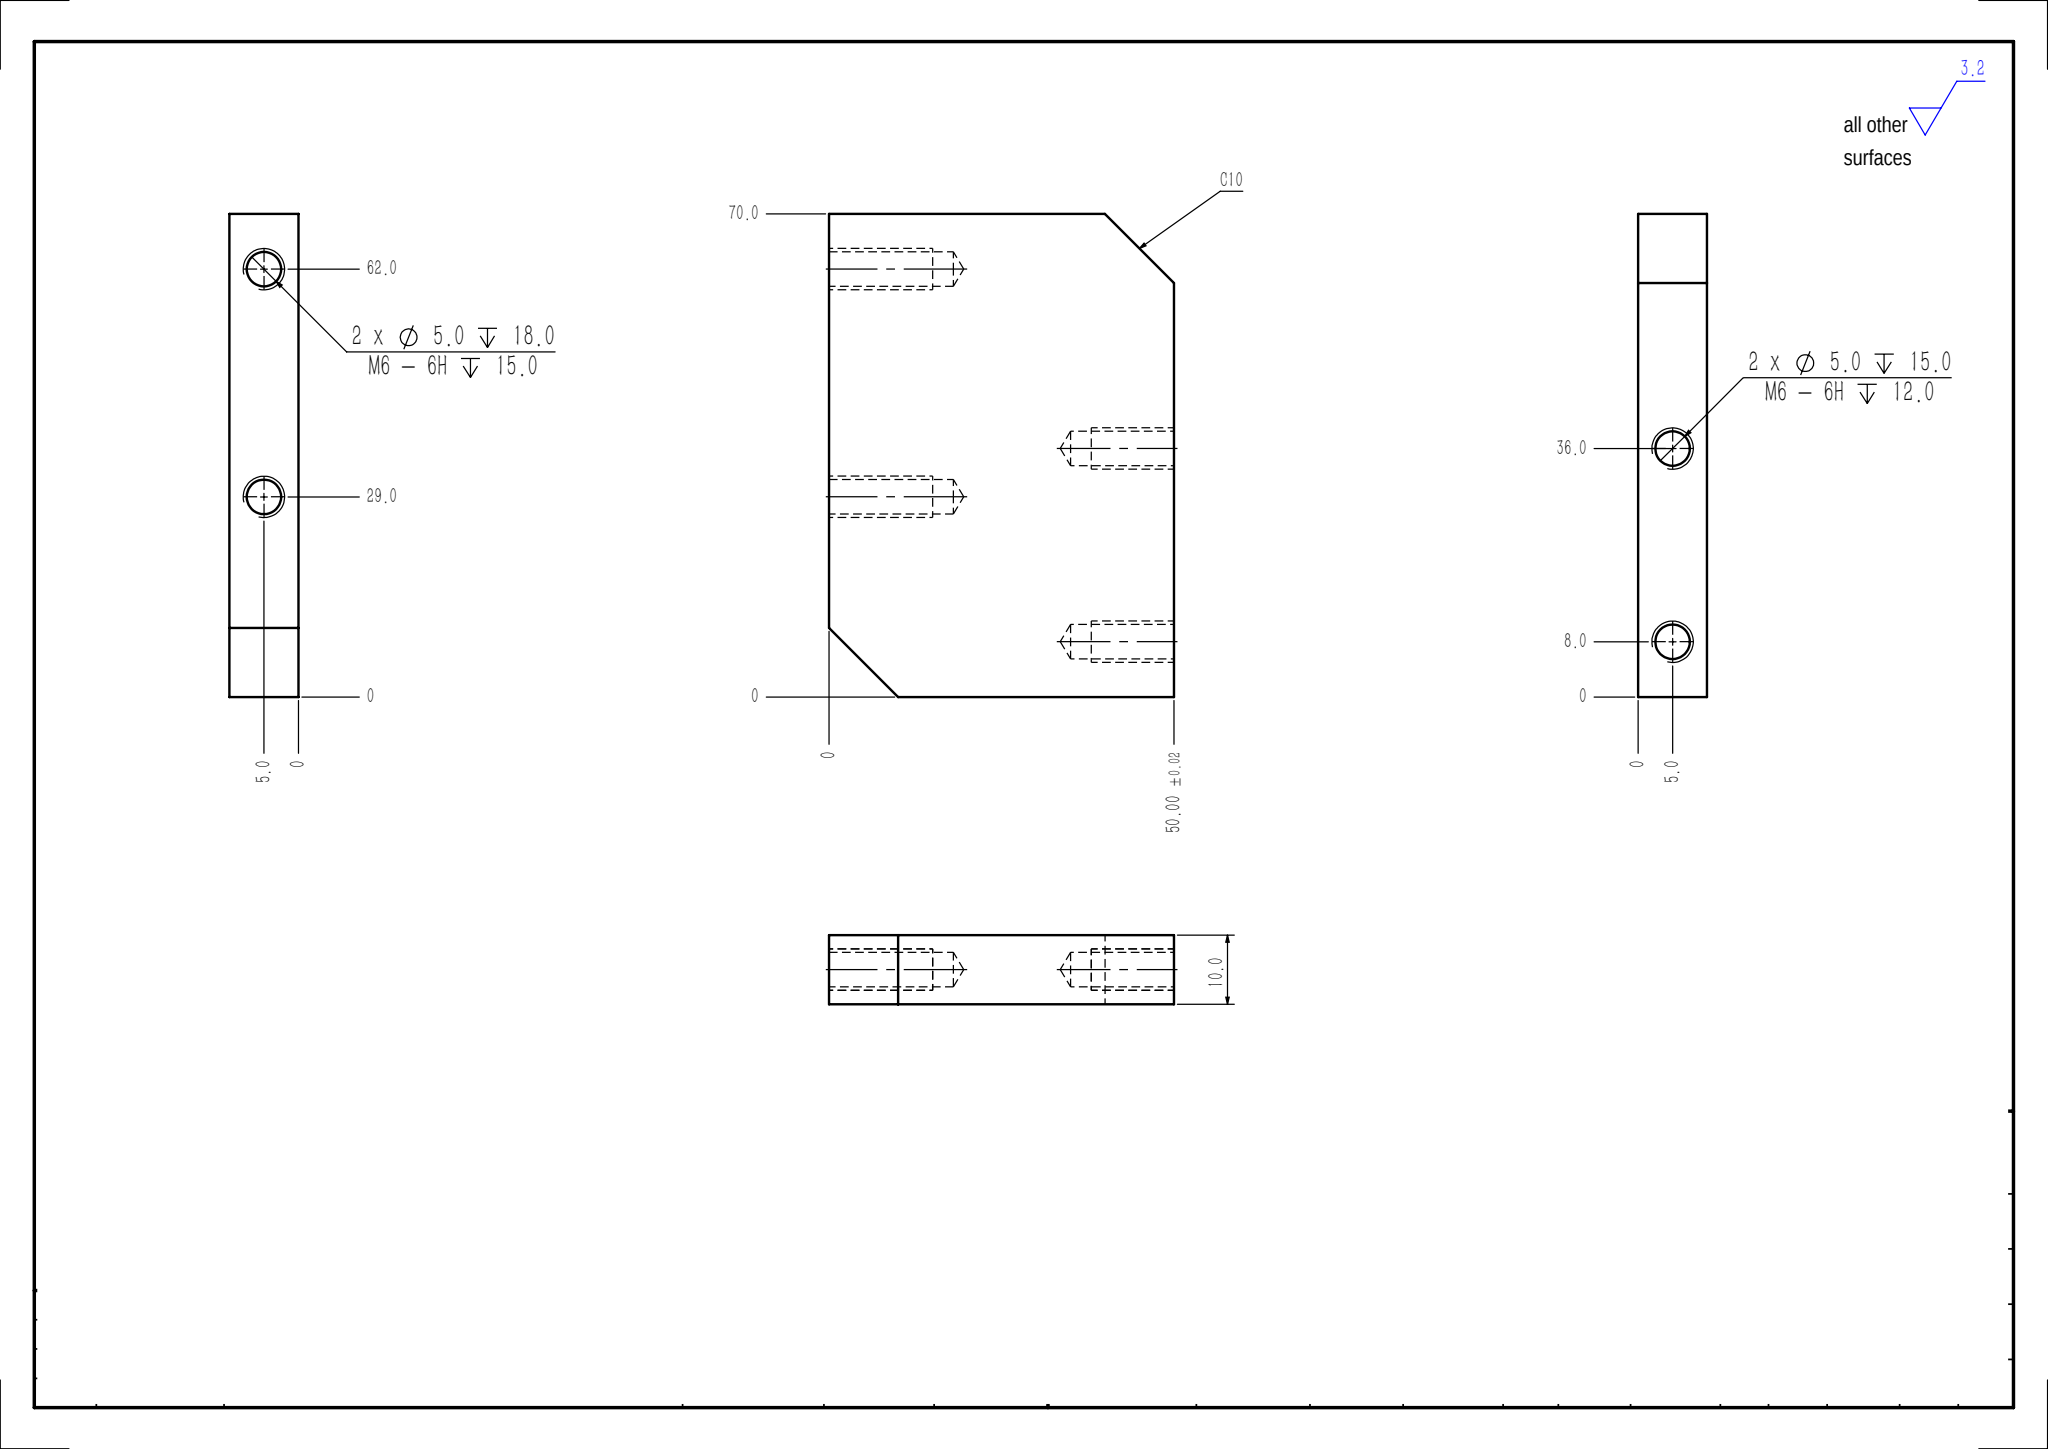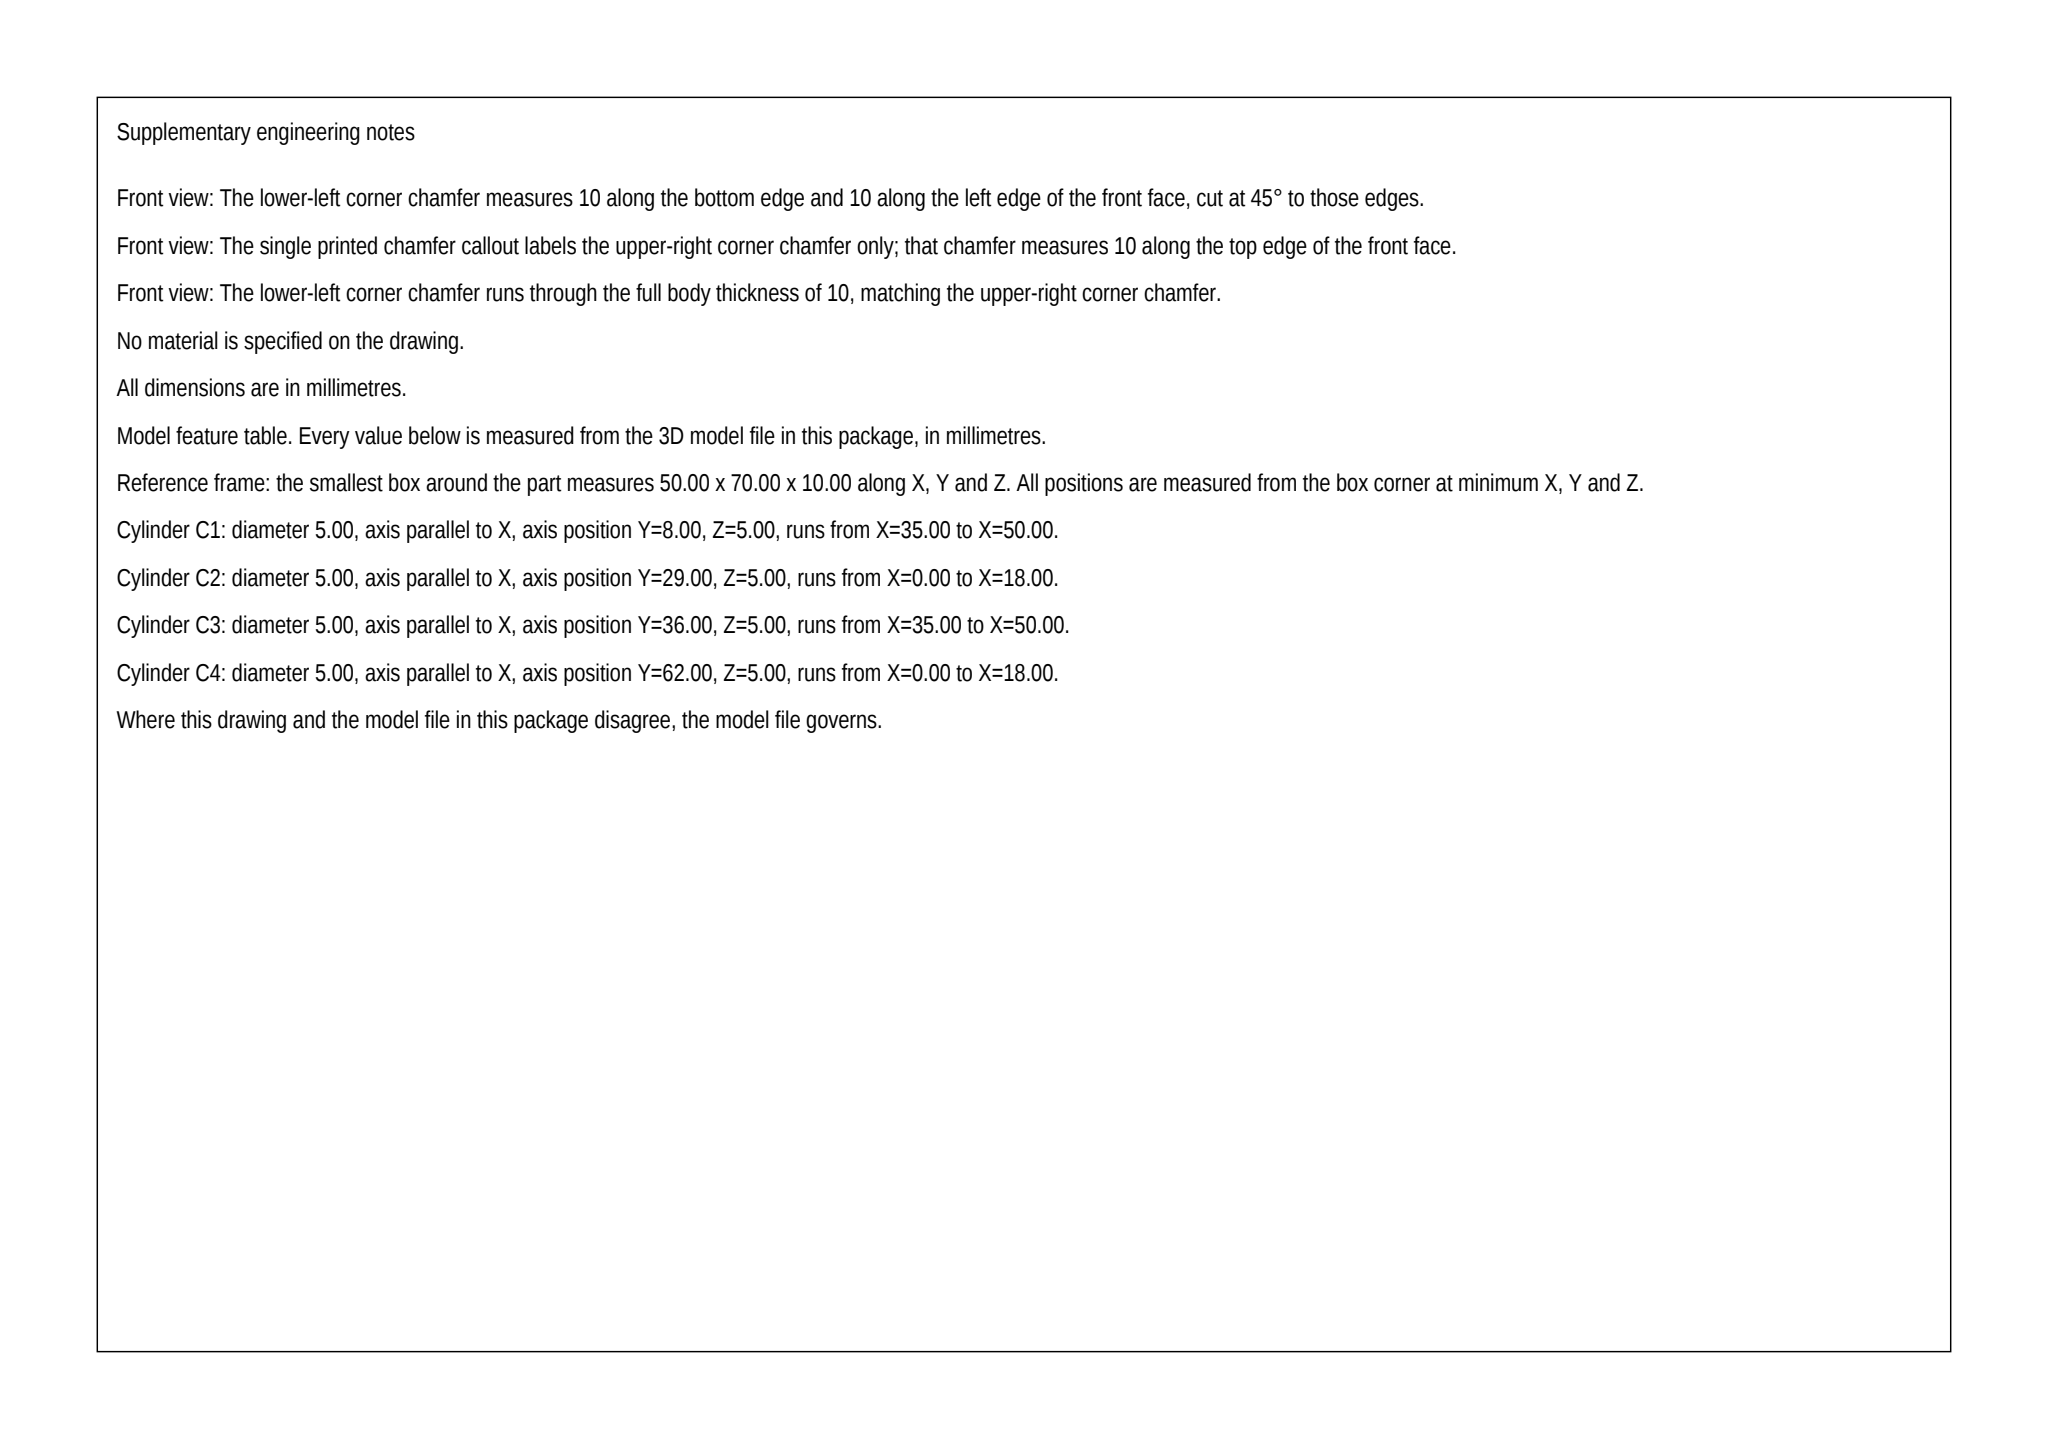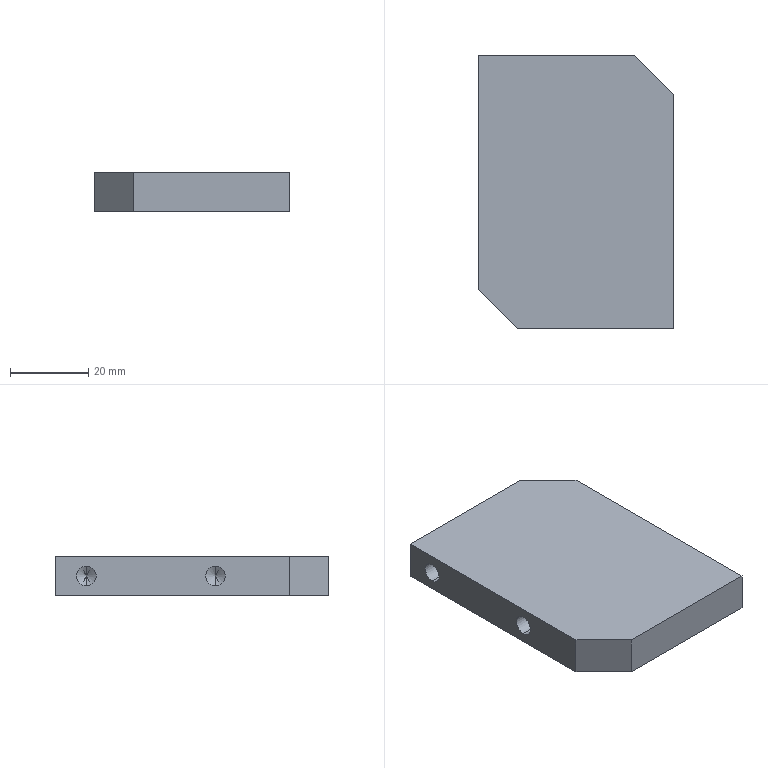Part | SolidWorks | mm | 1 solid | 24 faces | box 50 x 70 x 10 mm | volume 32665 mm3 | cylinder 8 | cone 8 | plane 8 | commonest cylinder face diameters 5 x8
Drawing notes:
C10 LOWER LEFT CORNER, FRONT VIEW (2X C10, 45 DEG) | from the solid: 50x70x10 bbox; lower-left corner cut 45 deg, 10 x 10 across corner, matching upper-right C10
2X C10 CHAMFER AT DIAG OPP CORNERS OF FRONT VIEW (TOP RH, BTM LH) | from the solid: inclined_planes: 45 deg faces, size 10x10x10, bbox_from [0,0,0] and [40,60,0] on 50x70x10 bbox
CHAMFERS FULL 10.0 THRU THICKNESS; NO OTHER CHAMFERS | from the solid: both inclined planes span z 0-10 (thickness 10.0); only 2 inclined planes in model
build123d program:
from build123d import *

# Parameters (mm, degrees)
SKETCH1_W             = 50
SKETCH1_H             = 70
BOSS_EXTRUDE1_DEPTH   = 10
M6_TAPPED_HOLE1_D     = 5
M6_TAPPED_HOLE1_DEPTH = 18
M6_TAPPED_HOLE1_TIP   = 1.502
M6_TAPPED_HOLE2_D     = 5
M6_TAPPED_HOLE2_DEPTH = 15
M6_TAPPED_HOLE2_TIP   = 1.502
CHAMFER1_SIZE         = 10


with BuildPart() as part:
    # Sketch1 → Boss-Extrude1 (new body)
    with BuildSketch(Plane.XY):
        Rectangle(SKETCH1_W, SKETCH1_H)
    extrude(amount=BOSS_EXTRUDE1_DEPTH)

    # M6 Tapped Hole1
    with Locations(Plane.ZY.offset(25)):
        with Locations((5, 27), (5, -6)):
            Hole(M6_TAPPED_HOLE1_D / 2, depth=M6_TAPPED_HOLE1_DEPTH)
            with Locations((0, 0, -(M6_TAPPED_HOLE1_DEPTH + M6_TAPPED_HOLE1_TIP / 2))):  # 118° drill point
                Cone(0, M6_TAPPED_HOLE1_D / 2, M6_TAPPED_HOLE1_TIP, mode=Mode.SUBTRACT)

    # M6 Tapped Hole2
    with Locations(Plane(origin=(25, 0, 0), x_dir=(0, 0, -1), z_dir=(1, 0, 0))):
        with Locations((-5, -27), (-5, 1)):
            Hole(M6_TAPPED_HOLE2_D / 2, depth=M6_TAPPED_HOLE2_DEPTH)
            with Locations((0, 0, -(M6_TAPPED_HOLE2_DEPTH + M6_TAPPED_HOLE2_TIP / 2))):  # 118° drill point
                Cone(0, M6_TAPPED_HOLE2_D / 2, M6_TAPPED_HOLE2_TIP, mode=Mode.SUBTRACT)

    # Chamfer1
    chamfer1_edges = [part.edges().sort_by_distance(p)[0] for p in [
        (-25, -35, 5),
        (25, 35, 5),
    ]]
    chamfer(chamfer1_edges, length=CHAMFER1_SIZE)


solid = part.part
STEP:
#1=CARTESIAN_POINT('',(10.,-27.,7.5));
#2=VERTEX_POINT('',#1);
#3=CARTESIAN_POINT('',(10.,-27.,2.5));
#4=VERTEX_POINT('',#3);
#5=CARTESIAN_POINT('',(10.,-27.,5.));
#6=DIRECTION('',(1.,0.,0.));
#7=DIRECTION('',(0.,0.,-1.));
#8=AXIS2_PLACEMENT_3D('',#5,#6,#7);
#9=CIRCLE('',#8,2.5);
#10=EDGE_CURVE('',#2,#4,#9,.T.);
#11=ORIENTED_EDGE('',*,*,#10,.F.);
#12=CARTESIAN_POINT('',(25.,-27.,7.5));
#13=VERTEX_POINT('',#12);
#14=CARTESIAN_POINT('',(25.,-27.,7.5));
#15=DIRECTION('',(1.,0.,0.));
#16=VECTOR('',#15,1000.);
#17=LINE('',#14,#16);
#18=EDGE_CURVE('',#2,#13,#17,.T.);
#19=ORIENTED_EDGE('',*,*,#18,.T.);
#20=CARTESIAN_POINT('',(25.,-27.,2.5));
#21=VERTEX_POINT('',#20);
#22=CARTESIAN_POINT('',(25.,-27.,5.));
#23=DIRECTION('',(1.,0.,0.));
#24=DIRECTION('',(0.,0.,-1.));
#25=AXIS2_PLACEMENT_3D('',#22,#23,#24);
#26=CIRCLE('',#25,2.5);
#27=EDGE_CURVE('',#13,#21,#26,.T.);
#28=ORIENTED_EDGE('',*,*,#27,.T.);
#29=CARTESIAN_POINT('',(25.,-27.,2.5));
#30=DIRECTION('',(1.,0.,0.));
#31=VECTOR('',#30,1000.);
#32=LINE('',#29,#31);
#33=EDGE_CURVE('',#4,#21,#32,.T.);
#34=ORIENTED_EDGE('',*,*,#33,.F.);
#35=EDGE_LOOP('',(#11,#19,#28,#34));
#36=FACE_OUTER_BOUND('',#35,.T.);
#37=CARTESIAN_POINT('',(25.,-27.,5.));
#38=DIRECTION('',(1.,0.,0.));
#39=DIRECTION('',(0.,0.,-1.));
#40=AXIS2_PLACEMENT_3D('',#37,#38,#39);
#41=CYLINDRICAL_SURFACE('',#40,2.5);
#42=ADVANCED_FACE('',(#36),#41,.F.);
#43=CARTESIAN_POINT('',(8.498,-27.,5.));
#44=VERTEX_POINT('',#43);
#45=CARTESIAN_POINT('',(10.,-27.,2.5));
#46=DIRECTION('',(0.515,0.,-0.8572));
#47=VECTOR('',#46,1000.);
#48=LINE('',#45,#47);
#49=EDGE_CURVE('',#44,#4,#48,.T.);
#50=ORIENTED_EDGE('',*,*,#49,.F.);
#51=CARTESIAN_POINT('',(10.,-27.,7.5));
#52=DIRECTION('',(0.515,0.,0.8572));
#53=VECTOR('',#52,1000.);
#54=LINE('',#51,#53);
#55=EDGE_CURVE('',#44,#2,#54,.T.);
#56=ORIENTED_EDGE('',*,*,#55,.T.);
#57=ORIENTED_EDGE('',*,*,#10,.T.);
#58=EDGE_LOOP('',(#50,#56,#57));
#59=FACE_OUTER_BOUND('',#58,.T.);
#60=CARTESIAN_POINT('',(10.,-27.,5.));
#61=DIRECTION('',(1.,0.,0.));
#62=DIRECTION('',(0.,0.,-1.));
#63=AXIS2_PLACEMENT_3D('',#60,#61,#62);
#64=CONICAL_SURFACE('',#63,2.5,1.03);
#65=ADVANCED_FACE('',(#59),#64,.F.);
#66=CARTESIAN_POINT('',(10.,1.,7.5));
#67=VERTEX_POINT('',#66);
#68=CARTESIAN_POINT('',(10.,1.,2.5));
#69=VERTEX_POINT('',#68);
#70=CARTESIAN_POINT('',(10.,1.,5.));
#71=DIRECTION('',(1.,0.,0.));
#72=DIRECTION('',(0.,0.,-1.));
#73=AXIS2_PLACEMENT_3D('',#70,#71,#72);
#74=CIRCLE('',#73,2.5);
#75=EDGE_CURVE('',#67,#69,#74,.T.);
#76=ORIENTED_EDGE('',*,*,#75,.F.);
#77=CARTESIAN_POINT('',(25.,1.,7.5));
#78=VERTEX_POINT('',#77);
#79=CARTESIAN_POINT('',(25.,1.,7.5));
#80=DIRECTION('',(1.,0.,0.));
#81=VECTOR('',#80,1000.);
#82=LINE('',#79,#81);
#83=EDGE_CURVE('',#67,#78,#82,.T.);
#84=ORIENTED_EDGE('',*,*,#83,.T.);
#85=CARTESIAN_POINT('',(25.,1.,2.5));
#86=VERTEX_POINT('',#85);
#87=CARTESIAN_POINT('',(25.,1.,5.));
#88=DIRECTION('',(1.,0.,0.));
#89=DIRECTION('',(0.,0.,-1.));
#90=AXIS2_PLACEMENT_3D('',#87,#88,#89);
#91=CIRCLE('',#90,2.5);
#92=EDGE_CURVE('',#78,#86,#91,.T.);
#93=ORIENTED_EDGE('',*,*,#92,.T.);
#94=CARTESIAN_POINT('',(25.,1.,2.5));
#95=DIRECTION('',(1.,0.,0.));
#96=VECTOR('',#95,1000.);
#97=LINE('',#94,#96);
#98=EDGE_CURVE('',#69,#86,#97,.T.);
#99=ORIENTED_EDGE('',*,*,#98,.F.);
#100=EDGE_LOOP('',(#76,#84,#93,#99));
#101=FACE_OUTER_BOUND('',#100,.T.);
#102=CARTESIAN_POINT('',(25.,1.,5.));
#103=DIRECTION('',(1.,0.,0.));
#104=DIRECTION('',(0.,0.,-1.));
#105=AXIS2_PLACEMENT_3D('',#102,#103,#104);
#106=CYLINDRICAL_SURFACE('',#105,2.5);
#107=ADVANCED_FACE('',(#101),#106,.F.);
#108=CARTESIAN_POINT('',(8.498,1.,5.));
#109=VERTEX_POINT('',#108);
#110=CARTESIAN_POINT('',(10.,1.,2.5));
#111=DIRECTION('',(0.515,0.,-0.8572));
#112=VECTOR('',#111,1000.);
#113=LINE('',#110,#112);
#114=EDGE_CURVE('',#109,#69,#113,.T.);
#115=ORIENTED_EDGE('',*,*,#114,.F.);
#116=CARTESIAN_POINT('',(10.,1.,7.5));
#117=DIRECTION('',(0.515,0.,0.8572));
#118=VECTOR('',#117,1000.);
#119=LINE('',#116,#118);
#120=EDGE_CURVE('',#109,#67,#119,.T.);
#121=ORIENTED_EDGE('',*,*,#120,.T.);
#122=ORIENTED_EDGE('',*,*,#75,.T.);
#123=EDGE_LOOP('',(#115,#121,#122));
#124=FACE_OUTER_BOUND('',#123,.T.);
#125=CARTESIAN_POINT('',(10.,1.,5.));
#126=DIRECTION('',(1.,0.,0.));
#127=DIRECTION('',(0.,0.,-1.));
#128=AXIS2_PLACEMENT_3D('',#125,#126,#127);
#129=CONICAL_SURFACE('',#128,2.5,1.03);
#130=ADVANCED_FACE('',(#124),#129,.F.);
#131=CARTESIAN_POINT('',(-7.,27.,2.5));
#132=VERTEX_POINT('',#131);
#133=CARTESIAN_POINT('',(-7.,27.,7.5));
#134=VERTEX_POINT('',#133);
#135=CARTESIAN_POINT('',(-7.,27.,5.));
#136=DIRECTION('',(-1.,0.,0.));
#137=DIRECTION('',(0.,0.,1.));
#138=AXIS2_PLACEMENT_3D('',#135,#136,#137);
#139=CIRCLE('',#138,2.5);
#140=EDGE_CURVE('',#132,#134,#139,.T.);
#141=ORIENTED_EDGE('',*,*,#140,.F.);
#142=CARTESIAN_POINT('',(-25.,27.,2.5));
#143=VERTEX_POINT('',#142);
#144=CARTESIAN_POINT('',(-25.,27.,2.5));
#145=DIRECTION('',(-1.,0.,0.));
#146=VECTOR('',#145,1000.);
#147=LINE('',#144,#146);
#148=EDGE_CURVE('',#132,#143,#147,.T.);
#149=ORIENTED_EDGE('',*,*,#148,.T.);
#150=CARTESIAN_POINT('',(-25.,27.,7.5));
#151=VERTEX_POINT('',#150);
#152=CARTESIAN_POINT('',(-25.,27.,5.));
#153=DIRECTION('',(-1.,0.,0.));
#154=DIRECTION('',(0.,0.,1.));
#155=AXIS2_PLACEMENT_3D('',#152,#153,#154);
#156=CIRCLE('',#155,2.5);
#157=EDGE_CURVE('',#143,#151,#156,.T.);
#158=ORIENTED_EDGE('',*,*,#157,.T.);
#159=CARTESIAN_POINT('',(-25.,27.,7.5));
#160=DIRECTION('',(-1.,0.,0.));
#161=VECTOR('',#160,1000.);
#162=LINE('',#159,#161);
#163=EDGE_CURVE('',#134,#151,#162,.T.);
#164=ORIENTED_EDGE('',*,*,#163,.F.);
#165=EDGE_LOOP('',(#141,#149,#158,#164));
#166=FACE_OUTER_BOUND('',#165,.T.);
#167=CARTESIAN_POINT('',(-25.,27.,5.));
#168=DIRECTION('',(-1.,0.,0.));
#169=DIRECTION('',(0.,0.,1.));
#170=AXIS2_PLACEMENT_3D('',#167,#168,#169);
#171=CYLINDRICAL_SURFACE('',#170,2.5);
#172=ADVANCED_FACE('',(#166),#171,.F.);
#173=CARTESIAN_POINT('',(-5.498,27.,5.));
#174=VERTEX_POINT('',#173);
#175=CARTESIAN_POINT('',(-7.,27.,7.5));
#176=DIRECTION('',(-0.515,0.,0.8572));
#177=VECTOR('',#176,1000.);
#178=LINE('',#175,#177);
#179=EDGE_CURVE('',#174,#134,#178,.T.);
#180=ORIENTED_EDGE('',*,*,#179,.F.);
#181=CARTESIAN_POINT('',(-7.,27.,2.5));
#182=DIRECTION('',(-0.515,0.,-0.8572));
#183=VECTOR('',#182,1000.);
#184=LINE('',#181,#183);
#185=EDGE_CURVE('',#174,#132,#184,.T.);
#186=ORIENTED_EDGE('',*,*,#185,.T.);
#187=ORIENTED_EDGE('',*,*,#140,.T.);
#188=EDGE_LOOP('',(#180,#186,#187));
#189=FACE_OUTER_BOUND('',#188,.T.);
#190=CARTESIAN_POINT('',(-7.,27.,5.));
#191=DIRECTION('',(-1.,0.,0.));
#192=DIRECTION('',(0.,0.,1.));
#193=AXIS2_PLACEMENT_3D('',#190,#191,#192);
#194=CONICAL_SURFACE('',#193,2.5,1.03);
#195=ADVANCED_FACE('',(#189),#194,.F.);
#196=CARTESIAN_POINT('',(-7.,-6.,2.5));
#197=VERTEX_POINT('',#196);
#198=CARTESIAN_POINT('',(-7.,-6.,7.5));
#199=VERTEX_POINT('',#198);
#200=CARTESIAN_POINT('',(-7.,-6.,5.));
#201=DIRECTION('',(-1.,0.,0.));
#202=DIRECTION('',(0.,0.,1.));
#203=AXIS2_PLACEMENT_3D('',#200,#201,#202);
#204=CIRCLE('',#203,2.5);
#205=EDGE_CURVE('',#197,#199,#204,.T.);
#206=ORIENTED_EDGE('',*,*,#205,.F.);
#207=CARTESIAN_POINT('',(-25.,-6.,2.5));
#208=VERTEX_POINT('',#207);
#209=CARTESIAN_POINT('',(-25.,-6.,2.5));
#210=DIRECTION('',(-1.,0.,0.));
#211=VECTOR('',#210,1000.);
#212=LINE('',#209,#211);
#213=EDGE_CURVE('',#197,#208,#212,.T.);
#214=ORIENTED_EDGE('',*,*,#213,.T.);
#215=CARTESIAN_POINT('',(-25.,-6.,7.5));
#216=VERTEX_POINT('',#215);
#217=CARTESIAN_POINT('',(-25.,-6.,5.));
#218=DIRECTION('',(-1.,0.,0.));
#219=DIRECTION('',(0.,0.,1.));
#220=AXIS2_PLACEMENT_3D('',#217,#218,#219);
#221=CIRCLE('',#220,2.5);
#222=EDGE_CURVE('',#208,#216,#221,.T.);
#223=ORIENTED_EDGE('',*,*,#222,.T.);
#224=CARTESIAN_POINT('',(-25.,-6.,7.5));
#225=DIRECTION('',(-1.,0.,0.));
#226=VECTOR('',#225,1000.);
#227=LINE('',#224,#226);
#228=EDGE_CURVE('',#199,#216,#227,.T.);
#229=ORIENTED_EDGE('',*,*,#228,.F.);
#230=EDGE_LOOP('',(#206,#214,#223,#229));
#231=FACE_OUTER_BOUND('',#230,.T.);
#232=CARTESIAN_POINT('',(-25.,-6.,5.));
#233=DIRECTION('',(-1.,0.,0.));
#234=DIRECTION('',(0.,0.,1.));
#235=AXIS2_PLACEMENT_3D('',#232,#233,#234);
#236=CYLINDRICAL_SURFACE('',#235,2.5);
#237=ADVANCED_FACE('',(#231),#236,.F.);
#238=CARTESIAN_POINT('',(-5.498,-6.,5.));
#239=VERTEX_POINT('',#238);
#240=CARTESIAN_POINT('',(-7.,-6.,7.5));
#241=DIRECTION('',(-0.515,0.,0.8572));
#242=VECTOR('',#241,1000.);
#243=LINE('',#240,#242);
#244=EDGE_CURVE('',#239,#199,#243,.T.);
#245=ORIENTED_EDGE('',*,*,#244,.F.);
#246=CARTESIAN_POINT('',(-7.,-6.,2.5));
#247=DIRECTION('',(-0.515,0.,-0.8572));
#248=VECTOR('',#247,1000.);
#249=LINE('',#246,#248);
#250=EDGE_CURVE('',#239,#197,#249,.T.);
#251=ORIENTED_EDGE('',*,*,#250,.T.);
#252=ORIENTED_EDGE('',*,*,#205,.T.);
#253=EDGE_LOOP('',(#245,#251,#252));
#254=FACE_OUTER_BOUND('',#253,.T.);
#255=CARTESIAN_POINT('',(-7.,-6.,5.));
#256=DIRECTION('',(-1.,0.,0.));
#257=DIRECTION('',(0.,0.,1.));
#258=AXIS2_PLACEMENT_3D('',#255,#256,#257);
#259=CONICAL_SURFACE('',#258,2.5,1.03);
#260=ADVANCED_FACE('',(#254),#259,.F.);
#261=CARTESIAN_POINT('',(25.,-27.,5.));
#262=DIRECTION('',(1.,0.,0.));
#263=DIRECTION('',(0.,0.,-1.));
#264=AXIS2_PLACEMENT_3D('',#261,#262,#263);
#265=CIRCLE('',#264,2.5);
#266=EDGE_CURVE('',#21,#13,#265,.T.);
#267=ORIENTED_EDGE('',*,*,#266,.F.);
#268=ORIENTED_EDGE('',*,*,#27,.F.);
#269=EDGE_LOOP('',(#267,#268));
#270=FACE_BOUND('',#269,.T.);
#271=CARTESIAN_POINT('',(25.,1.,5.));
#272=DIRECTION('',(1.,0.,0.));
#273=DIRECTION('',(0.,0.,-1.));
#274=AXIS2_PLACEMENT_3D('',#271,#272,#273);
#275=CIRCLE('',#274,2.5);
#276=EDGE_CURVE('',#86,#78,#275,.T.);
#277=ORIENTED_EDGE('',*,*,#276,.F.);
#278=ORIENTED_EDGE('',*,*,#92,.F.);
#279=EDGE_LOOP('',(#277,#278));
#280=FACE_BOUND('',#279,.T.);
#281=CARTESIAN_POINT('',(25.,-35.,0.));
#282=VERTEX_POINT('',#281);
#283=CARTESIAN_POINT('',(25.,25.,0.));
#284=VERTEX_POINT('',#283);
#285=CARTESIAN_POINT('',(25.,35.,0.));
#286=DIRECTION('',(-0.,1.,0.));
#287=VECTOR('',#286,1000.);
#288=LINE('',#285,#287);
#289=EDGE_CURVE('',#282,#284,#288,.T.);
#290=ORIENTED_EDGE('',*,*,#289,.T.);
#291=CARTESIAN_POINT('',(25.,25.,10.));
#292=VERTEX_POINT('',#291);
#293=CARTESIAN_POINT('',(25.,25.,10.));
#294=DIRECTION('',(0.,0.,1.));
#295=VECTOR('',#294,1000.);
#296=LINE('',#293,#295);
#297=EDGE_CURVE('',#284,#292,#296,.T.);
#298=ORIENTED_EDGE('',*,*,#297,.T.);
#299=CARTESIAN_POINT('',(25.,-35.,10.));
#300=VERTEX_POINT('',#299);
#301=CARTESIAN_POINT('',(25.,35.,10.));
#302=DIRECTION('',(-0.,1.,0.));
#303=VECTOR('',#302,1000.);
#304=LINE('',#301,#303);
#305=EDGE_CURVE('',#300,#292,#304,.T.);
#306=ORIENTED_EDGE('',*,*,#305,.F.);
#307=CARTESIAN_POINT('',(25.,-35.,10.));
#308=DIRECTION('',(0.,0.,-1.));
#309=VECTOR('',#308,1000.);
#310=LINE('',#307,#309);
#311=EDGE_CURVE('',#300,#282,#310,.T.);
#312=ORIENTED_EDGE('',*,*,#311,.T.);
#313=EDGE_LOOP('',(#290,#298,#306,#312));
#314=FACE_OUTER_BOUND('',#313,.T.);
#315=CARTESIAN_POINT('',(25.,35.,10.));
#316=DIRECTION('',(-1.,-0.,0.));
#317=DIRECTION('',(0.,-1.,0.));
#318=AXIS2_PLACEMENT_3D('',#315,#316,#317);
#319=PLANE('',#318);
#320=ADVANCED_FACE('',(#270,#280,#314),#319,.F.);
#321=CARTESIAN_POINT('',(15.,35.,10.));
#322=VERTEX_POINT('',#321);
#323=CARTESIAN_POINT('',(-25.,35.,10.));
#324=VERTEX_POINT('',#323);
#325=CARTESIAN_POINT('',(-25.,35.,10.));
#326=DIRECTION('',(-1.,0.,0.));
#327=VECTOR('',#326,1000.);
#328=LINE('',#325,#327);
#329=EDGE_CURVE('',#322,#324,#328,.T.);
#330=ORIENTED_EDGE('',*,*,#329,.F.);
#331=CARTESIAN_POINT('',(15.,35.,0.));
#332=VERTEX_POINT('',#331);
#333=CARTESIAN_POINT('',(15.,35.,10.));
#334=DIRECTION('',(0.,0.,-1.));
#335=VECTOR('',#334,1000.);
#336=LINE('',#333,#335);
#337=EDGE_CURVE('',#322,#332,#336,.T.);
#338=ORIENTED_EDGE('',*,*,#337,.T.);
#339=CARTESIAN_POINT('',(-25.,35.,0.));
#340=VERTEX_POINT('',#339);
#341=CARTESIAN_POINT('',(-25.,35.,0.));
#342=DIRECTION('',(-1.,0.,0.));
#343=VECTOR('',#342,1000.);
#344=LINE('',#341,#343);
#345=EDGE_CURVE('',#332,#340,#344,.T.);
#346=ORIENTED_EDGE('',*,*,#345,.T.);
#347=CARTESIAN_POINT('',(-25.,35.,10.));
#348=DIRECTION('',(0.,0.,-1.));
#349=VECTOR('',#348,1000.);
#350=LINE('',#347,#349);
#351=EDGE_CURVE('',#324,#340,#350,.T.);
#352=ORIENTED_EDGE('',*,*,#351,.F.);
#353=EDGE_LOOP('',(#330,#338,#346,#352));
#354=FACE_OUTER_BOUND('',#353,.T.);
#355=CARTESIAN_POINT('',(-25.,35.,10.));
#356=DIRECTION('',(0.,-1.,0.));
#357=DIRECTION('',(0.,0.,-1.));
#358=AXIS2_PLACEMENT_3D('',#355,#356,#357);
#359=PLANE('',#358);
#360=ADVANCED_FACE('',(#354),#359,.F.);
#361=CARTESIAN_POINT('',(-25.,27.,5.));
#362=DIRECTION('',(-1.,0.,0.));
#363=DIRECTION('',(0.,0.,1.));
#364=AXIS2_PLACEMENT_3D('',#361,#362,#363);
#365=CIRCLE('',#364,2.5);
#366=EDGE_CURVE('',#151,#143,#365,.T.);
#367=ORIENTED_EDGE('',*,*,#366,.F.);
#368=ORIENTED_EDGE('',*,*,#157,.F.);
#369=EDGE_LOOP('',(#367,#368));
#370=FACE_BOUND('',#369,.T.);
#371=CARTESIAN_POINT('',(-25.,-6.,5.));
#372=DIRECTION('',(-1.,0.,0.));
#373=DIRECTION('',(0.,0.,1.));
#374=AXIS2_PLACEMENT_3D('',#371,#372,#373);
#375=CIRCLE('',#374,2.5);
#376=EDGE_CURVE('',#216,#208,#375,.T.);
#377=ORIENTED_EDGE('',*,*,#376,.F.);
#378=ORIENTED_EDGE('',*,*,#222,.F.);
#379=EDGE_LOOP('',(#377,#378));
#380=FACE_BOUND('',#379,.T.);
#381=CARTESIAN_POINT('',(-25.,-25.,0.));
#382=VERTEX_POINT('',#381);
#383=CARTESIAN_POINT('',(-25.,35.,0.));
#384=DIRECTION('',(0.,-1.,0.));
#385=VECTOR('',#384,1000.);
#386=LINE('',#383,#385);
#387=EDGE_CURVE('',#340,#382,#386,.T.);
#388=ORIENTED_EDGE('',*,*,#387,.T.);
#389=CARTESIAN_POINT('',(-25.,-25.,10.));
#390=VERTEX_POINT('',#389);
#391=CARTESIAN_POINT('',(-25.,-25.,10.));
#392=DIRECTION('',(0.,0.,1.));
#393=VECTOR('',#392,1000.);
#394=LINE('',#391,#393);
#395=EDGE_CURVE('',#382,#390,#394,.T.);
#396=ORIENTED_EDGE('',*,*,#395,.T.);
#397=CARTESIAN_POINT('',(-25.,35.,10.));
#398=DIRECTION('',(0.,-1.,0.));
#399=VECTOR('',#398,1000.);
#400=LINE('',#397,#399);
#401=EDGE_CURVE('',#324,#390,#400,.T.);
#402=ORIENTED_EDGE('',*,*,#401,.F.);
#403=ORIENTED_EDGE('',*,*,#351,.T.);
#404=EDGE_LOOP('',(#388,#396,#402,#403));
#405=FACE_OUTER_BOUND('',#404,.T.);
#406=CARTESIAN_POINT('',(-25.,35.,10.));
#407=DIRECTION('',(1.,0.,0.));
#408=DIRECTION('',(-0.,1.,0.));
#409=AXIS2_PLACEMENT_3D('',#406,#407,#408);
#410=PLANE('',#409);
#411=ADVANCED_FACE('',(#370,#380,#405),#410,.F.);
#412=CARTESIAN_POINT('',(-15.,-35.,10.));
#413=VERTEX_POINT('',#412);
#414=CARTESIAN_POINT('',(-25.,-35.,10.));
#415=DIRECTION('',(1.,0.,0.));
#416=VECTOR('',#415,1000.);
#417=LINE('',#414,#416);
#418=EDGE_CURVE('',#413,#300,#417,.T.);
#419=ORIENTED_EDGE('',*,*,#418,.F.);
#420=CARTESIAN_POINT('',(-15.,-35.,0.));
#421=VERTEX_POINT('',#420);
#422=CARTESIAN_POINT('',(-15.,-35.,10.));
#423=DIRECTION('',(0.,0.,-1.));
#424=VECTOR('',#423,1000.);
#425=LINE('',#422,#424);
#426=EDGE_CURVE('',#413,#421,#425,.T.);
#427=ORIENTED_EDGE('',*,*,#426,.T.);
#428=CARTESIAN_POINT('',(-25.,-35.,0.));
#429=DIRECTION('',(1.,0.,0.));
#430=VECTOR('',#429,1000.);
#431=LINE('',#428,#430);
#432=EDGE_CURVE('',#421,#282,#431,.T.);
#433=ORIENTED_EDGE('',*,*,#432,.T.);
#434=ORIENTED_EDGE('',*,*,#311,.F.);
#435=EDGE_LOOP('',(#419,#427,#433,#434));
#436=FACE_OUTER_BOUND('',#435,.T.);
#437=CARTESIAN_POINT('',(-25.,-35.,10.));
#438=DIRECTION('',(0.,1.,0.));
#439=DIRECTION('',(0.,0.,1.));
#440=AXIS2_PLACEMENT_3D('',#437,#438,#439);
#441=PLANE('',#440);
#442=ADVANCED_FACE('',(#436),#441,.F.);
#443=ORIENTED_EDGE('',*,*,#305,.T.);
#444=CARTESIAN_POINT('',(25.,25.,10.));
#445=DIRECTION('',(-0.7071,0.7071,0.));
#446=VECTOR('',#445,1000.);
#447=LINE('',#444,#446);
#448=EDGE_CURVE('',#292,#322,#447,.T.);
#449=ORIENTED_EDGE('',*,*,#448,.T.);
#450=ORIENTED_EDGE('',*,*,#329,.T.);
#451=ORIENTED_EDGE('',*,*,#401,.T.);
#452=CARTESIAN_POINT('',(-25.,-25.,10.));
#453=DIRECTION('',(0.7071,-0.7071,0.));
#454=VECTOR('',#453,1000.);
#455=LINE('',#452,#454);
#456=EDGE_CURVE('',#390,#413,#455,.T.);
#457=ORIENTED_EDGE('',*,*,#456,.T.);
#458=ORIENTED_EDGE('',*,*,#418,.T.);
#459=EDGE_LOOP('',(#443,#449,#450,#451,#457,#458));
#460=FACE_OUTER_BOUND('',#459,.T.);
#461=CARTESIAN_POINT('',(0.,0.,10.));
#462=DIRECTION('',(0.,0.,1.));
#463=DIRECTION('',(1.,0.,0.));
#464=AXIS2_PLACEMENT_3D('',#461,#462,#463);
#465=PLANE('',#464);
#466=ADVANCED_FACE('',(#460),#465,.T.);
#467=ORIENTED_EDGE('',*,*,#345,.F.);
#468=CARTESIAN_POINT('',(15.,35.,0.));
#469=DIRECTION('',(0.7071,-0.7071,0.));
#470=VECTOR('',#469,1000.);
#471=LINE('',#468,#470);
#472=EDGE_CURVE('',#332,#284,#471,.T.);
#473=ORIENTED_EDGE('',*,*,#472,.T.);
#474=ORIENTED_EDGE('',*,*,#289,.F.);
#475=ORIENTED_EDGE('',*,*,#432,.F.);
#476=CARTESIAN_POINT('',(-15.,-35.,0.));
#477=DIRECTION('',(-0.7071,0.7071,0.));
#478=VECTOR('',#477,1000.);
#479=LINE('',#476,#478);
#480=EDGE_CURVE('',#421,#382,#479,.T.);
#481=ORIENTED_EDGE('',*,*,#480,.T.);
#482=ORIENTED_EDGE('',*,*,#387,.F.);
#483=EDGE_LOOP('',(#467,#473,#474,#475,#481,#482));
#484=FACE_OUTER_BOUND('',#483,.T.);
#485=CARTESIAN_POINT('',(0.,0.,0.));
#486=DIRECTION('',(0.,0.,1.));
#487=DIRECTION('',(1.,0.,0.));
#488=AXIS2_PLACEMENT_3D('',#485,#486,#487);
#489=PLANE('',#488);
#490=ADVANCED_FACE('',(#484),#489,.F.);
#491=ORIENTED_EDGE('',*,*,#250,.F.);
#492=ORIENTED_EDGE('',*,*,#244,.T.);
#493=CARTESIAN_POINT('',(-7.,-6.,5.));
#494=DIRECTION('',(-1.,0.,0.));
#495=DIRECTION('',(0.,0.,1.));
#496=AXIS2_PLACEMENT_3D('',#493,#494,#495);
#497=CIRCLE('',#496,2.5);
#498=EDGE_CURVE('',#199,#197,#497,.T.);
#499=ORIENTED_EDGE('',*,*,#498,.T.);
#500=EDGE_LOOP('',(#491,#492,#499));
#501=FACE_OUTER_BOUND('',#500,.T.);
#502=CARTESIAN_POINT('',(-7.,-6.,5.));
#503=DIRECTION('',(-1.,0.,0.));
#504=DIRECTION('',(0.,0.,1.));
#505=AXIS2_PLACEMENT_3D('',#502,#503,#504);
#506=CONICAL_SURFACE('',#505,2.5,1.03);
#507=ADVANCED_FACE('',(#501),#506,.F.);
#508=ORIENTED_EDGE('',*,*,#213,.F.);
#509=ORIENTED_EDGE('',*,*,#498,.F.);
#510=ORIENTED_EDGE('',*,*,#228,.T.);
#511=ORIENTED_EDGE('',*,*,#376,.T.);
#512=EDGE_LOOP('',(#508,#509,#510,#511));
#513=FACE_OUTER_BOUND('',#512,.T.);
#514=CARTESIAN_POINT('',(-25.,-6.,5.));
#515=DIRECTION('',(-1.,0.,0.));
#516=DIRECTION('',(0.,0.,1.));
#517=AXIS2_PLACEMENT_3D('',#514,#515,#516);
#518=CYLINDRICAL_SURFACE('',#517,2.5);
#519=ADVANCED_FACE('',(#513),#518,.F.);
#520=ORIENTED_EDGE('',*,*,#185,.F.);
#521=ORIENTED_EDGE('',*,*,#179,.T.);
#522=CARTESIAN_POINT('',(-7.,27.,5.));
#523=DIRECTION('',(-1.,0.,0.));
#524=DIRECTION('',(0.,0.,1.));
#525=AXIS2_PLACEMENT_3D('',#522,#523,#524);
#526=CIRCLE('',#525,2.5);
#527=EDGE_CURVE('',#134,#132,#526,.T.);
#528=ORIENTED_EDGE('',*,*,#527,.T.);
#529=EDGE_LOOP('',(#520,#521,#528));
#530=FACE_OUTER_BOUND('',#529,.T.);
#531=CARTESIAN_POINT('',(-7.,27.,5.));
#532=DIRECTION('',(-1.,0.,0.));
#533=DIRECTION('',(0.,0.,1.));
#534=AXIS2_PLACEMENT_3D('',#531,#532,#533);
#535=CONICAL_SURFACE('',#534,2.5,1.03);
#536=ADVANCED_FACE('',(#530),#535,.F.);
#537=ORIENTED_EDGE('',*,*,#148,.F.);
#538=ORIENTED_EDGE('',*,*,#527,.F.);
#539=ORIENTED_EDGE('',*,*,#163,.T.);
#540=ORIENTED_EDGE('',*,*,#366,.T.);
#541=EDGE_LOOP('',(#537,#538,#539,#540));
#542=FACE_OUTER_BOUND('',#541,.T.);
#543=CARTESIAN_POINT('',(-25.,27.,5.));
#544=DIRECTION('',(-1.,0.,0.));
#545=DIRECTION('',(0.,0.,1.));
#546=AXIS2_PLACEMENT_3D('',#543,#544,#545);
#547=CYLINDRICAL_SURFACE('',#546,2.5);
#548=ADVANCED_FACE('',(#542),#547,.F.);
#549=ORIENTED_EDGE('',*,*,#120,.F.);
#550=ORIENTED_EDGE('',*,*,#114,.T.);
#551=CARTESIAN_POINT('',(10.,1.,5.));
#552=DIRECTION('',(1.,0.,0.));
#553=DIRECTION('',(0.,0.,-1.));
#554=AXIS2_PLACEMENT_3D('',#551,#552,#553);
#555=CIRCLE('',#554,2.5);
#556=EDGE_CURVE('',#69,#67,#555,.T.);
#557=ORIENTED_EDGE('',*,*,#556,.T.);
#558=EDGE_LOOP('',(#549,#550,#557));
#559=FACE_OUTER_BOUND('',#558,.T.);
#560=CARTESIAN_POINT('',(10.,1.,5.));
#561=DIRECTION('',(1.,0.,0.));
#562=DIRECTION('',(0.,0.,-1.));
#563=AXIS2_PLACEMENT_3D('',#560,#561,#562);
#564=CONICAL_SURFACE('',#563,2.5,1.03);
#565=ADVANCED_FACE('',(#559),#564,.F.);
#566=ORIENTED_EDGE('',*,*,#83,.F.);
#567=ORIENTED_EDGE('',*,*,#556,.F.);
#568=ORIENTED_EDGE('',*,*,#98,.T.);
#569=ORIENTED_EDGE('',*,*,#276,.T.);
#570=EDGE_LOOP('',(#566,#567,#568,#569));
#571=FACE_OUTER_BOUND('',#570,.T.);
#572=CARTESIAN_POINT('',(25.,1.,5.));
#573=DIRECTION('',(1.,0.,0.));
#574=DIRECTION('',(0.,0.,-1.));
#575=AXIS2_PLACEMENT_3D('',#572,#573,#574);
#576=CYLINDRICAL_SURFACE('',#575,2.5);
#577=ADVANCED_FACE('',(#571),#576,.F.);
#578=ORIENTED_EDGE('',*,*,#55,.F.);
#579=ORIENTED_EDGE('',*,*,#49,.T.);
#580=CARTESIAN_POINT('',(10.,-27.,5.));
#581=DIRECTION('',(1.,0.,0.));
#582=DIRECTION('',(0.,0.,-1.));
#583=AXIS2_PLACEMENT_3D('',#580,#581,#582);
#584=CIRCLE('',#583,2.5);
#585=EDGE_CURVE('',#4,#2,#584,.T.);
#586=ORIENTED_EDGE('',*,*,#585,.T.);
#587=EDGE_LOOP('',(#578,#579,#586));
#588=FACE_OUTER_BOUND('',#587,.T.);
#589=CARTESIAN_POINT('',(10.,-27.,5.));
#590=DIRECTION('',(1.,0.,0.));
#591=DIRECTION('',(0.,0.,-1.));
#592=AXIS2_PLACEMENT_3D('',#589,#590,#591);
#593=CONICAL_SURFACE('',#592,2.5,1.03);
#594=ADVANCED_FACE('',(#588),#593,.F.);
#595=ORIENTED_EDGE('',*,*,#18,.F.);
#596=ORIENTED_EDGE('',*,*,#585,.F.);
#597=ORIENTED_EDGE('',*,*,#33,.T.);
#598=ORIENTED_EDGE('',*,*,#266,.T.);
#599=EDGE_LOOP('',(#595,#596,#597,#598));
#600=FACE_OUTER_BOUND('',#599,.T.);
#601=CARTESIAN_POINT('',(25.,-27.,5.));
#602=DIRECTION('',(1.,0.,0.));
#603=DIRECTION('',(0.,0.,-1.));
#604=AXIS2_PLACEMENT_3D('',#601,#602,#603);
#605=CYLINDRICAL_SURFACE('',#604,2.5);
#606=ADVANCED_FACE('',(#600),#605,.F.);
#607=ORIENTED_EDGE('',*,*,#448,.F.);
#608=ORIENTED_EDGE('',*,*,#297,.F.);
#609=ORIENTED_EDGE('',*,*,#472,.F.);
#610=ORIENTED_EDGE('',*,*,#337,.F.);
#611=EDGE_LOOP('',(#607,#608,#609,#610));
#612=FACE_OUTER_BOUND('',#611,.T.);
#613=CARTESIAN_POINT('',(15.,35.,10.));
#614=DIRECTION('',(-0.7071,-0.7071,0.));
#615=DIRECTION('',(0.,0.,-1.));
#616=AXIS2_PLACEMENT_3D('',#613,#614,#615);
#617=PLANE('',#616);
#618=ADVANCED_FACE('',(#612),#617,.F.);
#619=ORIENTED_EDGE('',*,*,#456,.F.);
#620=ORIENTED_EDGE('',*,*,#395,.F.);
#621=ORIENTED_EDGE('',*,*,#480,.F.);
#622=ORIENTED_EDGE('',*,*,#426,.F.);
#623=EDGE_LOOP('',(#619,#620,#621,#622));
#624=FACE_OUTER_BOUND('',#623,.T.);
#625=CARTESIAN_POINT('',(-15.,-35.,10.));
#626=DIRECTION('',(0.7071,0.7071,0.));
#627=DIRECTION('',(0.,0.,-1.));
#628=AXIS2_PLACEMENT_3D('',#625,#626,#627);
#629=PLANE('',#628);
#630=ADVANCED_FACE('',(#624),#629,.F.);
#631=CLOSED_SHELL('',(#42,#65,#107,#130,#172,#195,#237,#260,#320,#360,#411,#442,#466,#490,#507,#519,#536,#548,#565,#577,#594,#606,#618,#630));
#632=MANIFOLD_SOLID_BREP('',#631);
#633=CARTESIAN_POINT('',(0.,0.,0.));
#634=DIRECTION('',(0.,0.,1.));
#635=DIRECTION('',(1.,0.,0.));
#636=AXIS2_PLACEMENT_3D('',#633,#634,#635);
#637=(LENGTH_UNIT()NAMED_UNIT(*)SI_UNIT(.MILLI.,.METRE.));
#638=UNCERTAINTY_MEASURE_WITH_UNIT(LENGTH_MEASURE(0.00001),#637,'','');
#639=(NAMED_UNIT(*)PLANE_ANGLE_UNIT()SI_UNIT($,.RADIAN.));
#640=(NAMED_UNIT(*)SI_UNIT($,.STERADIAN.)SOLID_ANGLE_UNIT());
#641=(GEOMETRIC_REPRESENTATION_CONTEXT(3)GLOBAL_UNCERTAINTY_ASSIGNED_CONTEXT((#638))GLOBAL_UNIT_ASSIGNED_CONTEXT((#637,#639,#640))REPRESENTATION_CONTEXT('',''));
#642=ADVANCED_BREP_SHAPE_REPRESENTATION('',(#632,#636),#641);